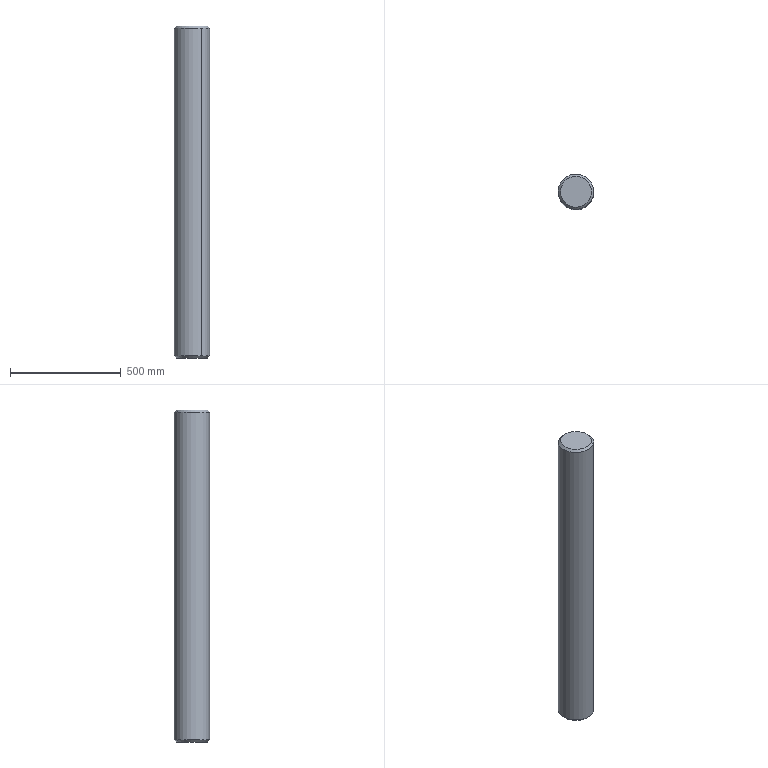Component | SolidWorks | WheelMandrel-1 | 1 solid | 8 faces | box 160 x 160 x 1500 mm | volume 30111118 mm3 | cone 4 | cylinder 2 | plane 2 | commonest cylinder face diameters 160 x2 | material 45
build123d program:
from build123d import *

# Parameters (mm, degrees)
SKETCH1_R           = 80
BOSS_EXTRUDE1_DEPTH = 1500
CHAMFER1_SIZE       = 10


with BuildPart() as part:
    # Sketch1 → Boss-Extrude1 (new body)
    with BuildSketch(Plane.XY):
        with Locations((1138.564, 280.356)):
            Circle(SKETCH1_R)
    extrude(amount=BOSS_EXTRUDE1_DEPTH)

    # Chamfer1
    chamfer1_edges = [part.edges().sort_by_distance(p)[0] for p in [
        (1058.564, 280.356, 0),
        (1058.564, 280.356, 1500),
    ]]
    chamfer(chamfer1_edges, length=CHAMFER1_SIZE)


solid = part.part

# Placed as in the assembly
solid = solid.moved(Location((0, 0, -255), (0, 0, 0)))
STEP:
#1=COLOUR_RGB('',0.7922,0.8196,0.9333);
#2=FILL_AREA_STYLE_COLOUR('',#1);
#3=FILL_AREA_STYLE('',(#2));
#4=SURFACE_STYLE_FILL_AREA(#3);
#5=SURFACE_SIDE_STYLE('',(#4));
#6=SURFACE_STYLE_USAGE(.BOTH.,#5);
#7=PRESENTATION_STYLE_ASSIGNMENT((#6));
#8=CARTESIAN_POINT('',(43.35,13.365,-10.039));
#9=VERTEX_POINT('',#8);
#10=CARTESIAN_POINT('',(46.301,8.71,-10.039));
#11=VERTEX_POINT('',#10);
#12=CARTESIAN_POINT('',(44.825,11.038,-10.039));
#13=DIRECTION('',(0.,0.,-1.));
#14=DIRECTION('',(-0.5353,0.8447,0.));
#15=AXIS2_PLACEMENT_3D('',#12,#13,#14);
#16=CIRCLE('',#15,2.756);
#17=EDGE_CURVE('',#9,#11,#16,.T.);
#18=ORIENTED_EDGE('',*,*,#17,.F.);
#19=CARTESIAN_POINT('',(43.139,13.698,-9.646));
#20=VERTEX_POINT('',#19);
#21=CARTESIAN_POINT('',(43.35,13.365,-10.039));
#22=DIRECTION('',(-0.3785,0.5973,0.7071));
#23=VECTOR('',#22,39.37);
#24=LINE('',#21,#23);
#25=EDGE_CURVE('',#9,#20,#24,.T.);
#26=ORIENTED_EDGE('',*,*,#25,.T.);
#27=CARTESIAN_POINT('',(46.511,8.377,-9.646));
#28=VERTEX_POINT('',#27);
#29=CARTESIAN_POINT('',(44.825,11.038,-9.646));
#30=DIRECTION('',(0.,0.,1.));
#31=DIRECTION('',(-0.5353,0.8447,0.));
#32=AXIS2_PLACEMENT_3D('',#29,#30,#31);
#33=CIRCLE('',#32,3.15);
#34=EDGE_CURVE('',#28,#20,#33,.T.);
#35=ORIENTED_EDGE('',*,*,#34,.F.);
#36=CARTESIAN_POINT('',(46.301,8.71,-10.039));
#37=DIRECTION('',(0.3785,-0.5973,0.7071));
#38=VECTOR('',#37,39.37);
#39=LINE('',#36,#38);
#40=EDGE_CURVE('',#11,#28,#39,.T.);
#41=ORIENTED_EDGE('',*,*,#40,.F.);
#42=EDGE_LOOP('',(#18,#26,#35,#41));
#43=FACE_OUTER_BOUND('',#42,.T.);
#44=CARTESIAN_POINT('',(44.825,11.038,-10.039));
#45=DIRECTION('',(0.,0.,1.));
#46=DIRECTION('',(0.5353,-0.8447,0.));
#47=AXIS2_PLACEMENT_3D('',#44,#45,#46);
#48=CONICAL_SURFACE('',#47,2.756,0.7854);
#49=ADVANCED_FACE('',(#43),#48,.T.);
#50=CARTESIAN_POINT('',(46.301,8.71,49.016));
#51=VERTEX_POINT('',#50);
#52=CARTESIAN_POINT('',(43.35,13.365,49.016));
#53=VERTEX_POINT('',#52);
#54=CARTESIAN_POINT('',(44.825,11.038,49.016));
#55=DIRECTION('',(0.,0.,1.));
#56=DIRECTION('',(-0.5353,0.8447,0.));
#57=AXIS2_PLACEMENT_3D('',#54,#55,#56);
#58=CIRCLE('',#57,2.756);
#59=EDGE_CURVE('',#51,#53,#58,.T.);
#60=ORIENTED_EDGE('',*,*,#59,.F.);
#61=CARTESIAN_POINT('',(46.511,8.377,48.622));
#62=VERTEX_POINT('',#61);
#63=CARTESIAN_POINT('',(46.511,8.377,48.622));
#64=DIRECTION('',(0.3785,-0.5973,-0.7071));
#65=VECTOR('',#64,39.37);
#66=LINE('',#63,#65);
#67=EDGE_CURVE('',#51,#62,#66,.T.);
#68=ORIENTED_EDGE('',*,*,#67,.T.);
#69=CARTESIAN_POINT('',(43.139,13.698,48.622));
#70=VERTEX_POINT('',#69);
#71=CARTESIAN_POINT('',(44.825,11.038,48.622));
#72=DIRECTION('',(0.,0.,-1.));
#73=DIRECTION('',(-0.5353,0.8447,0.));
#74=AXIS2_PLACEMENT_3D('',#71,#72,#73);
#75=CIRCLE('',#74,3.15);
#76=EDGE_CURVE('',#70,#62,#75,.T.);
#77=ORIENTED_EDGE('',*,*,#76,.F.);
#78=CARTESIAN_POINT('',(43.139,13.698,48.622));
#79=DIRECTION('',(-0.3785,0.5973,-0.7071));
#80=VECTOR('',#79,39.37);
#81=LINE('',#78,#80);
#82=EDGE_CURVE('',#53,#70,#81,.T.);
#83=ORIENTED_EDGE('',*,*,#82,.F.);
#84=EDGE_LOOP('',(#60,#68,#77,#83));
#85=FACE_OUTER_BOUND('',#84,.T.);
#86=CARTESIAN_POINT('',(44.825,11.038,48.622));
#87=DIRECTION('',(0.,0.,-1.));
#88=DIRECTION('',(-0.5353,0.8447,0.));
#89=AXIS2_PLACEMENT_3D('',#86,#87,#88);
#90=CONICAL_SURFACE('',#89,3.15,0.7854);
#91=ADVANCED_FACE('',(#85),#90,.T.);
#92=ORIENTED_EDGE('',*,*,#34,.T.);
#93=CARTESIAN_POINT('',(43.139,13.698,-10.039));
#94=DIRECTION('',(0.,0.,1.));
#95=VECTOR('',#94,39.37);
#96=LINE('',#93,#95);
#97=EDGE_CURVE('',#20,#70,#96,.T.);
#98=ORIENTED_EDGE('',*,*,#97,.T.);
#99=ORIENTED_EDGE('',*,*,#76,.T.);
#100=CARTESIAN_POINT('',(46.511,8.377,-10.039));
#101=DIRECTION('',(0.,0.,1.));
#102=VECTOR('',#101,39.37);
#103=LINE('',#100,#102);
#104=EDGE_CURVE('',#28,#62,#103,.T.);
#105=ORIENTED_EDGE('',*,*,#104,.F.);
#106=EDGE_LOOP('',(#92,#98,#99,#105));
#107=FACE_OUTER_BOUND('',#106,.T.);
#108=CARTESIAN_POINT('',(44.825,11.038,-10.039));
#109=DIRECTION('',(0.,0.,1.));
#110=DIRECTION('',(0.5353,-0.8447,0.));
#111=AXIS2_PLACEMENT_3D('',#108,#109,#110);
#112=CYLINDRICAL_SURFACE('',#111,3.15);
#113=ADVANCED_FACE('',(#107),#112,.T.);
#114=ORIENTED_EDGE('',*,*,#97,.F.);
#115=CARTESIAN_POINT('',(44.825,11.038,-9.646));
#116=DIRECTION('',(0.,0.,1.));
#117=DIRECTION('',(-0.5353,0.8447,0.));
#118=AXIS2_PLACEMENT_3D('',#115,#116,#117);
#119=CIRCLE('',#118,3.15);
#120=EDGE_CURVE('',#20,#28,#119,.T.);
#121=ORIENTED_EDGE('',*,*,#120,.T.);
#122=ORIENTED_EDGE('',*,*,#104,.T.);
#123=CARTESIAN_POINT('',(44.825,11.038,48.622));
#124=DIRECTION('',(0.,0.,-1.));
#125=DIRECTION('',(-0.5353,0.8447,0.));
#126=AXIS2_PLACEMENT_3D('',#123,#124,#125);
#127=CIRCLE('',#126,3.15);
#128=EDGE_CURVE('',#62,#70,#127,.T.);
#129=ORIENTED_EDGE('',*,*,#128,.T.);
#130=EDGE_LOOP('',(#114,#121,#122,#129));
#131=FACE_OUTER_BOUND('',#130,.T.);
#132=CARTESIAN_POINT('',(44.825,11.038,-10.039));
#133=DIRECTION('',(0.,0.,1.));
#134=DIRECTION('',(0.5353,-0.8447,0.));
#135=AXIS2_PLACEMENT_3D('',#132,#133,#134);
#136=CYLINDRICAL_SURFACE('',#135,3.15);
#137=ADVANCED_FACE('',(#131),#136,.T.);
#138=CARTESIAN_POINT('',(44.825,11.038,-10.039));
#139=DIRECTION('',(0.,0.,-1.));
#140=DIRECTION('',(-0.5353,0.8447,0.));
#141=AXIS2_PLACEMENT_3D('',#138,#139,#140);
#142=CIRCLE('',#141,2.756);
#143=EDGE_CURVE('',#11,#9,#142,.T.);
#144=ORIENTED_EDGE('',*,*,#143,.T.);
#145=ORIENTED_EDGE('',*,*,#17,.T.);
#146=EDGE_LOOP('',(#144,#145));
#147=FACE_OUTER_BOUND('',#146,.T.);
#148=CARTESIAN_POINT('',(44.825,11.038,-10.039));
#149=DIRECTION('',(0.,0.,-1.));
#150=DIRECTION('',(-0.5353,0.8447,0.));
#151=AXIS2_PLACEMENT_3D('',#148,#149,#150);
#152=PLANE('',#151);
#153=ADVANCED_FACE('',(#147),#152,.T.);
#154=CARTESIAN_POINT('',(44.825,11.038,49.016));
#155=DIRECTION('',(0.,0.,1.));
#156=DIRECTION('',(-0.5353,0.8447,0.));
#157=AXIS2_PLACEMENT_3D('',#154,#155,#156);
#158=CIRCLE('',#157,2.756);
#159=EDGE_CURVE('',#53,#51,#158,.T.);
#160=ORIENTED_EDGE('',*,*,#159,.T.);
#161=ORIENTED_EDGE('',*,*,#59,.T.);
#162=EDGE_LOOP('',(#160,#161));
#163=FACE_OUTER_BOUND('',#162,.T.);
#164=CARTESIAN_POINT('',(44.825,11.038,49.016));
#165=DIRECTION('',(0.,0.,-1.));
#166=DIRECTION('',(-0.5353,0.8447,0.));
#167=AXIS2_PLACEMENT_3D('',#164,#165,#166);
#168=PLANE('',#167);
#169=ADVANCED_FACE('',(#163),#168,.F.);
#170=ORIENTED_EDGE('',*,*,#67,.F.);
#171=ORIENTED_EDGE('',*,*,#159,.F.);
#172=ORIENTED_EDGE('',*,*,#82,.T.);
#173=ORIENTED_EDGE('',*,*,#128,.F.);
#174=EDGE_LOOP('',(#170,#171,#172,#173));
#175=FACE_OUTER_BOUND('',#174,.T.);
#176=CARTESIAN_POINT('',(44.825,11.038,48.622));
#177=DIRECTION('',(0.,0.,-1.));
#178=DIRECTION('',(-0.5353,0.8447,0.));
#179=AXIS2_PLACEMENT_3D('',#176,#177,#178);
#180=CONICAL_SURFACE('',#179,3.15,0.7854);
#181=ADVANCED_FACE('',(#175),#180,.T.);
#182=ORIENTED_EDGE('',*,*,#25,.F.);
#183=ORIENTED_EDGE('',*,*,#143,.F.);
#184=ORIENTED_EDGE('',*,*,#40,.T.);
#185=ORIENTED_EDGE('',*,*,#120,.F.);
#186=EDGE_LOOP('',(#182,#183,#184,#185));
#187=FACE_OUTER_BOUND('',#186,.T.);
#188=CARTESIAN_POINT('',(44.825,11.038,-10.039));
#189=DIRECTION('',(0.,0.,1.));
#190=DIRECTION('',(0.5353,-0.8447,0.));
#191=AXIS2_PLACEMENT_3D('',#188,#189,#190);
#192=CONICAL_SURFACE('',#191,2.756,0.7854);
#193=ADVANCED_FACE('',(#187),#192,.T.);
#194=CLOSED_SHELL('',(#49,#91,#113,#137,#153,#169,#181,#193));
#195=MANIFOLD_SOLID_BREP('',#194);
#196=STYLED_ITEM('',(#7),#195);
#197=(LENGTH_UNIT()NAMED_UNIT(*)SI_UNIT($,.METRE.));
#198=LENGTH_MEASURE_WITH_UNIT(LENGTH_MEASURE(0.0254),#197);
#199=DIMENSIONAL_EXPONENTS(1.,0.,0.,0.,0.,0.,0.);
#200=(CONVERSION_BASED_UNIT('',#198)LENGTH_UNIT()NAMED_UNIT(#199));
#201=UNCERTAINTY_MEASURE_WITH_UNIT(LENGTH_MEASURE(0.00001),#200,'','');
#202=(NAMED_UNIT(*)PLANE_ANGLE_UNIT()SI_UNIT($,.RADIAN.));
#203=(NAMED_UNIT(*)SI_UNIT($,.STERADIAN.)SOLID_ANGLE_UNIT());
#204=(GEOMETRIC_REPRESENTATION_CONTEXT(3)GLOBAL_UNCERTAINTY_ASSIGNED_CONTEXT((#201))GLOBAL_UNIT_ASSIGNED_CONTEXT((#200,#202,#203))REPRESENTATION_CONTEXT('',''));
#205=MECHANICAL_DESIGN_GEOMETRIC_PRESENTATION_REPRESENTATION('',(#196),#204);
#206=PRESENTATION_LAYER_ASSIGNMENT('','',(#196));
#207=CARTESIAN_POINT('',(0.,0.,0.));
#208=DIRECTION('',(0.,0.,1.));
#209=DIRECTION('',(1.,0.,0.));
#210=AXIS2_PLACEMENT_3D('',#207,#208,#209);
#211=(LENGTH_UNIT()NAMED_UNIT(*)SI_UNIT($,.METRE.));
#212=LENGTH_MEASURE_WITH_UNIT(LENGTH_MEASURE(0.0254),#211);
#213=DIMENSIONAL_EXPONENTS(1.,0.,0.,0.,0.,0.,0.);
#214=(CONVERSION_BASED_UNIT('',#212)LENGTH_UNIT()NAMED_UNIT(#213));
#215=UNCERTAINTY_MEASURE_WITH_UNIT(LENGTH_MEASURE(0.00001),#214,'','');
#216=(NAMED_UNIT(*)PLANE_ANGLE_UNIT()SI_UNIT($,.RADIAN.));
#217=(NAMED_UNIT(*)SI_UNIT($,.STERADIAN.)SOLID_ANGLE_UNIT());
#218=(GEOMETRIC_REPRESENTATION_CONTEXT(3)GLOBAL_UNCERTAINTY_ASSIGNED_CONTEXT((#215))GLOBAL_UNIT_ASSIGNED_CONTEXT((#214,#216,#217))REPRESENTATION_CONTEXT('',''));
#219=ADVANCED_BREP_SHAPE_REPRESENTATION('',(#195,#210),#218);